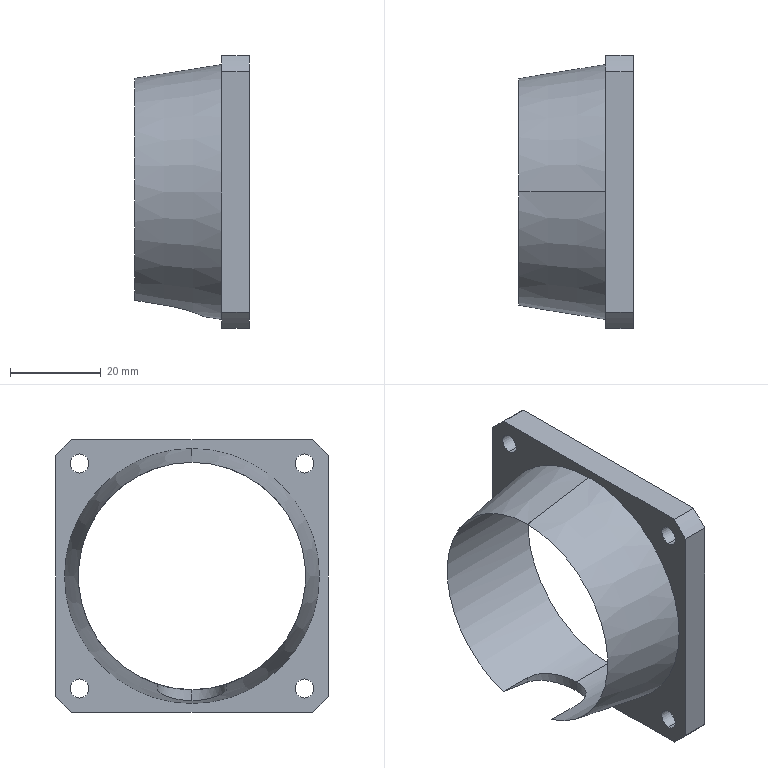Component | SolidWorks | DoubleFilmTransport-1_Connector-1 | 1 solid | 34 faces | volume 13864 mm3 | cylinder 16 | cone 10 | plane 8 | commonest cylinder face diameters 4.2 x8 80 x4 15 x2 50 x2